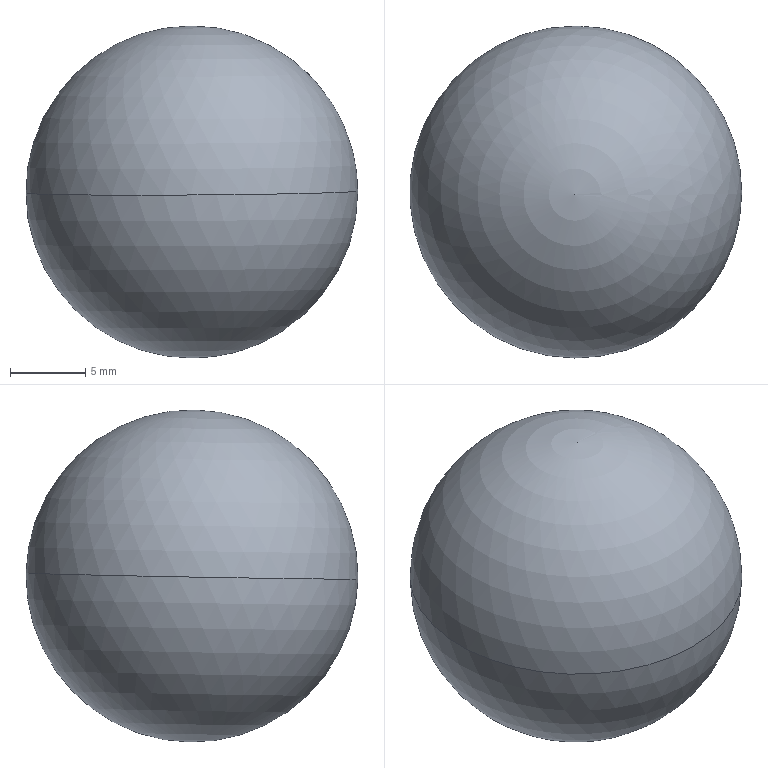Component | SolidWorks | 216InnerTubeAssembly-1_WaterSeparatorBall-1 | 1 solid | 2 faces | box 22 x 22 x 22 mm | volume 5575 mm3 | sphere 2 | material Alloy Steel
build123d program:
from build123d import *
from build123d.topology import SkipClean


with BuildPart() as part:
    # Sketch1 → Revolve2 (revolve)
    with SkipClean():  # the faces are left unmerged after this step: merging them gives an invalid solid
        with BuildSketch(Plane.XY):
            with BuildLine():
                ThreePointArc((11, 0), (7.778, 7.778), (0, 11))
                Line((0, 11), (0, -11))
                ThreePointArc((0, -11), (7.778, -7.778), (11, 0))
            make_face()
            with BuildLine():
                Line((0, -11), (0, 11))
                ThreePointArc((0, 11), (-11, 0), (0, -11))
            make_face()
        revolve(axis=Axis((0, 11, 0), (0, -1, 0)))


solid = part.part

# Placed as in the assembly
solid = solid.moved(Location((1160.457, 0.5043, 0.1044), (0, 0, 0)))
STEP:
#1=CARTESIAN_POINT('',(45.685,-0.4131,-0.003672));
#2=VERTEX_POINT('',#1);
#3=CARTESIAN_POINT('',(45.69,0.4528,0.0119));
#4=VERTEX_POINT('',#3);
#5=CARTESIAN_POINT('',(45.687,0.01985,0.004112));
#6=DIRECTION('',(-0.006333,-0.01794,0.9998));
#7=DIRECTION('',(0.,-0.9998,-0.01794));
#8=AXIS2_PLACEMENT_3D('',#5,#6,#7);
#9=CIRCLE('',#8,0.4331);
#10=EDGE_CURVE('',#2,#4,#9,.T.);
#11=ORIENTED_EDGE('',*,*,#10,.F.);
#12=CARTESIAN_POINT('',(45.687,0.01985,0.004112));
#13=DIRECTION('',(0.006333,0.01794,-0.9998));
#14=DIRECTION('',(0.,0.9998,0.01794));
#15=AXIS2_PLACEMENT_3D('',#12,#13,#14);
#16=CIRCLE('',#15,0.4331);
#17=EDGE_CURVE('',#2,#4,#16,.T.);
#18=ORIENTED_EDGE('',*,*,#17,.T.);
#19=EDGE_LOOP('',(#11,#18));
#20=FACE_OUTER_BOUND('',#19,.T.);
#21=CARTESIAN_POINT('',(45.687,0.01985,0.004112));
#22=DIRECTION('',(0.006333,0.01794,-0.9998));
#23=DIRECTION('',(1.,-0.006106,0.006225));
#24=AXIS2_PLACEMENT_3D('',#21,#22,#23);
#25=SPHERICAL_SURFACE('',#24,0.4331);
#26=ADVANCED_FACE('',(#20),#25,.T.);
#27=ORIENTED_EDGE('',*,*,#17,.F.);
#28=ORIENTED_EDGE('',*,*,#10,.T.);
#29=EDGE_LOOP('',(#27,#28));
#30=FACE_OUTER_BOUND('',#29,.T.);
#31=CARTESIAN_POINT('',(45.687,0.01985,0.004112));
#32=DIRECTION('',(0.006333,0.01794,-0.9998));
#33=DIRECTION('',(1.,-0.006106,0.006225));
#34=AXIS2_PLACEMENT_3D('',#31,#32,#33);
#35=SPHERICAL_SURFACE('',#34,0.4331);
#36=ADVANCED_FACE('',(#30),#35,.T.);
#37=CLOSED_SHELL('',(#26,#36));
#38=MANIFOLD_SOLID_BREP('',#37);
#39=CARTESIAN_POINT('',(0.,0.,0.));
#40=DIRECTION('',(0.,0.,1.));
#41=DIRECTION('',(1.,0.,0.));
#42=AXIS2_PLACEMENT_3D('',#39,#40,#41);
#43=(LENGTH_UNIT()NAMED_UNIT(*)SI_UNIT($,.METRE.));
#44=LENGTH_MEASURE_WITH_UNIT(LENGTH_MEASURE(0.0254),#43);
#45=DIMENSIONAL_EXPONENTS(1.,0.,0.,0.,0.,0.,0.);
#46=(CONVERSION_BASED_UNIT('',#44)LENGTH_UNIT()NAMED_UNIT(#45));
#47=UNCERTAINTY_MEASURE_WITH_UNIT(LENGTH_MEASURE(0.00001),#46,'','');
#48=(NAMED_UNIT(*)PLANE_ANGLE_UNIT()SI_UNIT($,.RADIAN.));
#49=(NAMED_UNIT(*)SI_UNIT($,.STERADIAN.)SOLID_ANGLE_UNIT());
#50=(GEOMETRIC_REPRESENTATION_CONTEXT(3)GLOBAL_UNCERTAINTY_ASSIGNED_CONTEXT((#47))GLOBAL_UNIT_ASSIGNED_CONTEXT((#46,#48,#49))REPRESENTATION_CONTEXT('',''));
#51=ADVANCED_BREP_SHAPE_REPRESENTATION('',(#38,#42),#50);
#52=COLOUR_RGB('',0.7922,0.8196,0.9333);
#53=FILL_AREA_STYLE_COLOUR('',#52);
#54=FILL_AREA_STYLE('',(#53));
#55=SURFACE_STYLE_FILL_AREA(#54);
#56=SURFACE_SIDE_STYLE('',(#55));
#57=SURFACE_STYLE_USAGE(.BOTH.,#56);
#58=PRESENTATION_STYLE_ASSIGNMENT((#57));
#59=STYLED_ITEM('',(#58),#38);
#60=(LENGTH_UNIT()NAMED_UNIT(*)SI_UNIT($,.METRE.));
#61=LENGTH_MEASURE_WITH_UNIT(LENGTH_MEASURE(0.0254),#60);
#62=DIMENSIONAL_EXPONENTS(1.,0.,0.,0.,0.,0.,0.);
#63=(CONVERSION_BASED_UNIT('',#61)LENGTH_UNIT()NAMED_UNIT(#62));
#64=UNCERTAINTY_MEASURE_WITH_UNIT(LENGTH_MEASURE(0.00001),#63,'','');
#65=(NAMED_UNIT(*)PLANE_ANGLE_UNIT()SI_UNIT($,.RADIAN.));
#66=(NAMED_UNIT(*)SI_UNIT($,.STERADIAN.)SOLID_ANGLE_UNIT());
#67=(GEOMETRIC_REPRESENTATION_CONTEXT(3)GLOBAL_UNCERTAINTY_ASSIGNED_CONTEXT((#64))GLOBAL_UNIT_ASSIGNED_CONTEXT((#63,#65,#66))REPRESENTATION_CONTEXT('',''));
#68=MECHANICAL_DESIGN_GEOMETRIC_PRESENTATION_REPRESENTATION('',(#59),#67);
#69=PRESENTATION_LAYER_ASSIGNMENT('','',(#59));